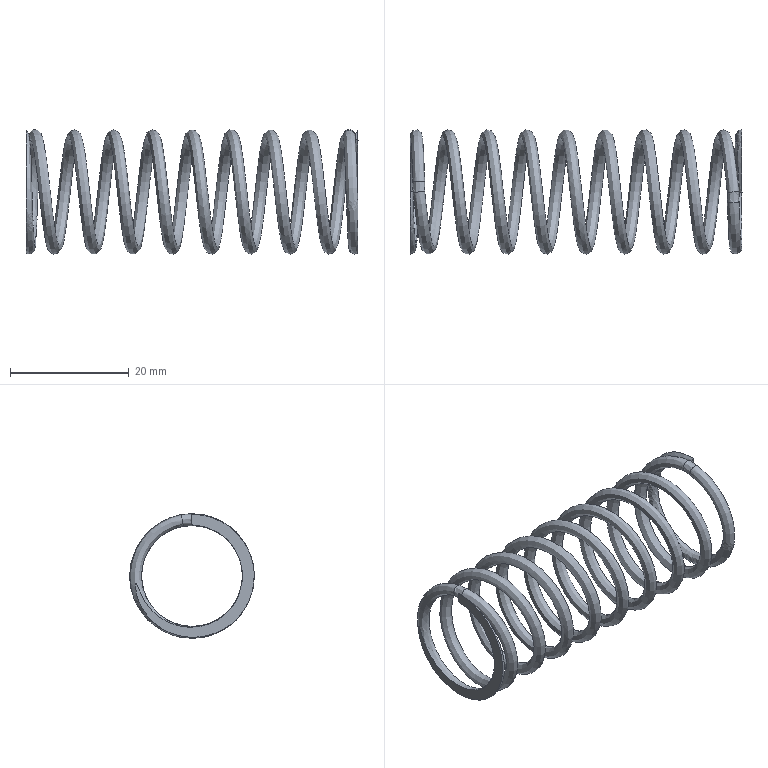Component | NX | SPRING_CYLINDER_COMPRESSION_1 | 1 solid | 9 faces | volume 1748 mm3 | spline 5 | plane 4